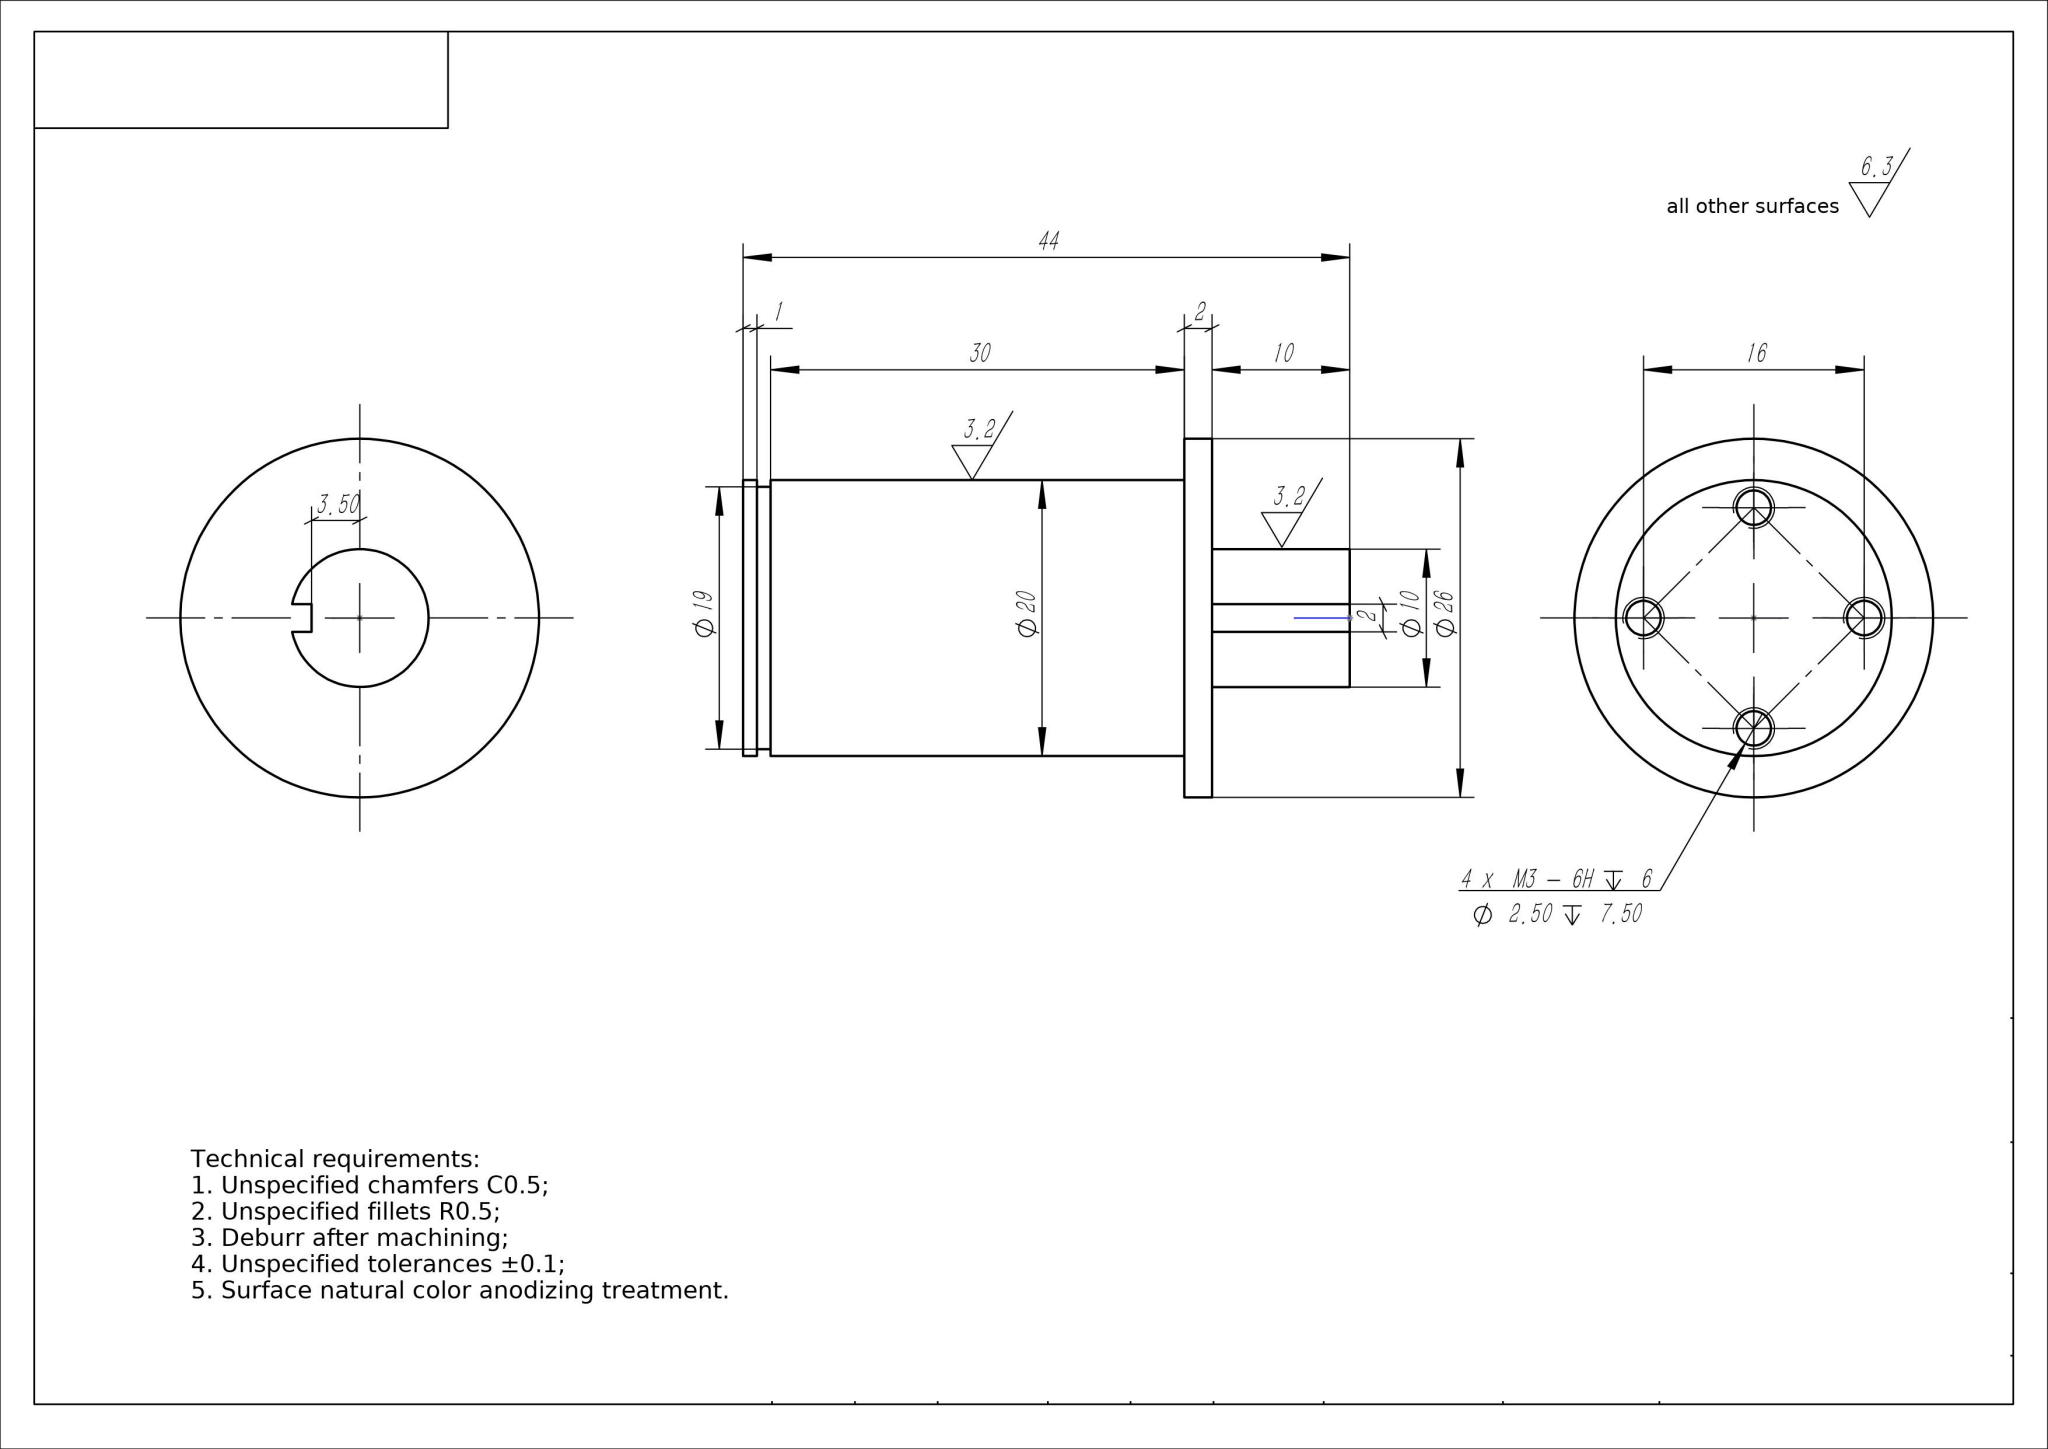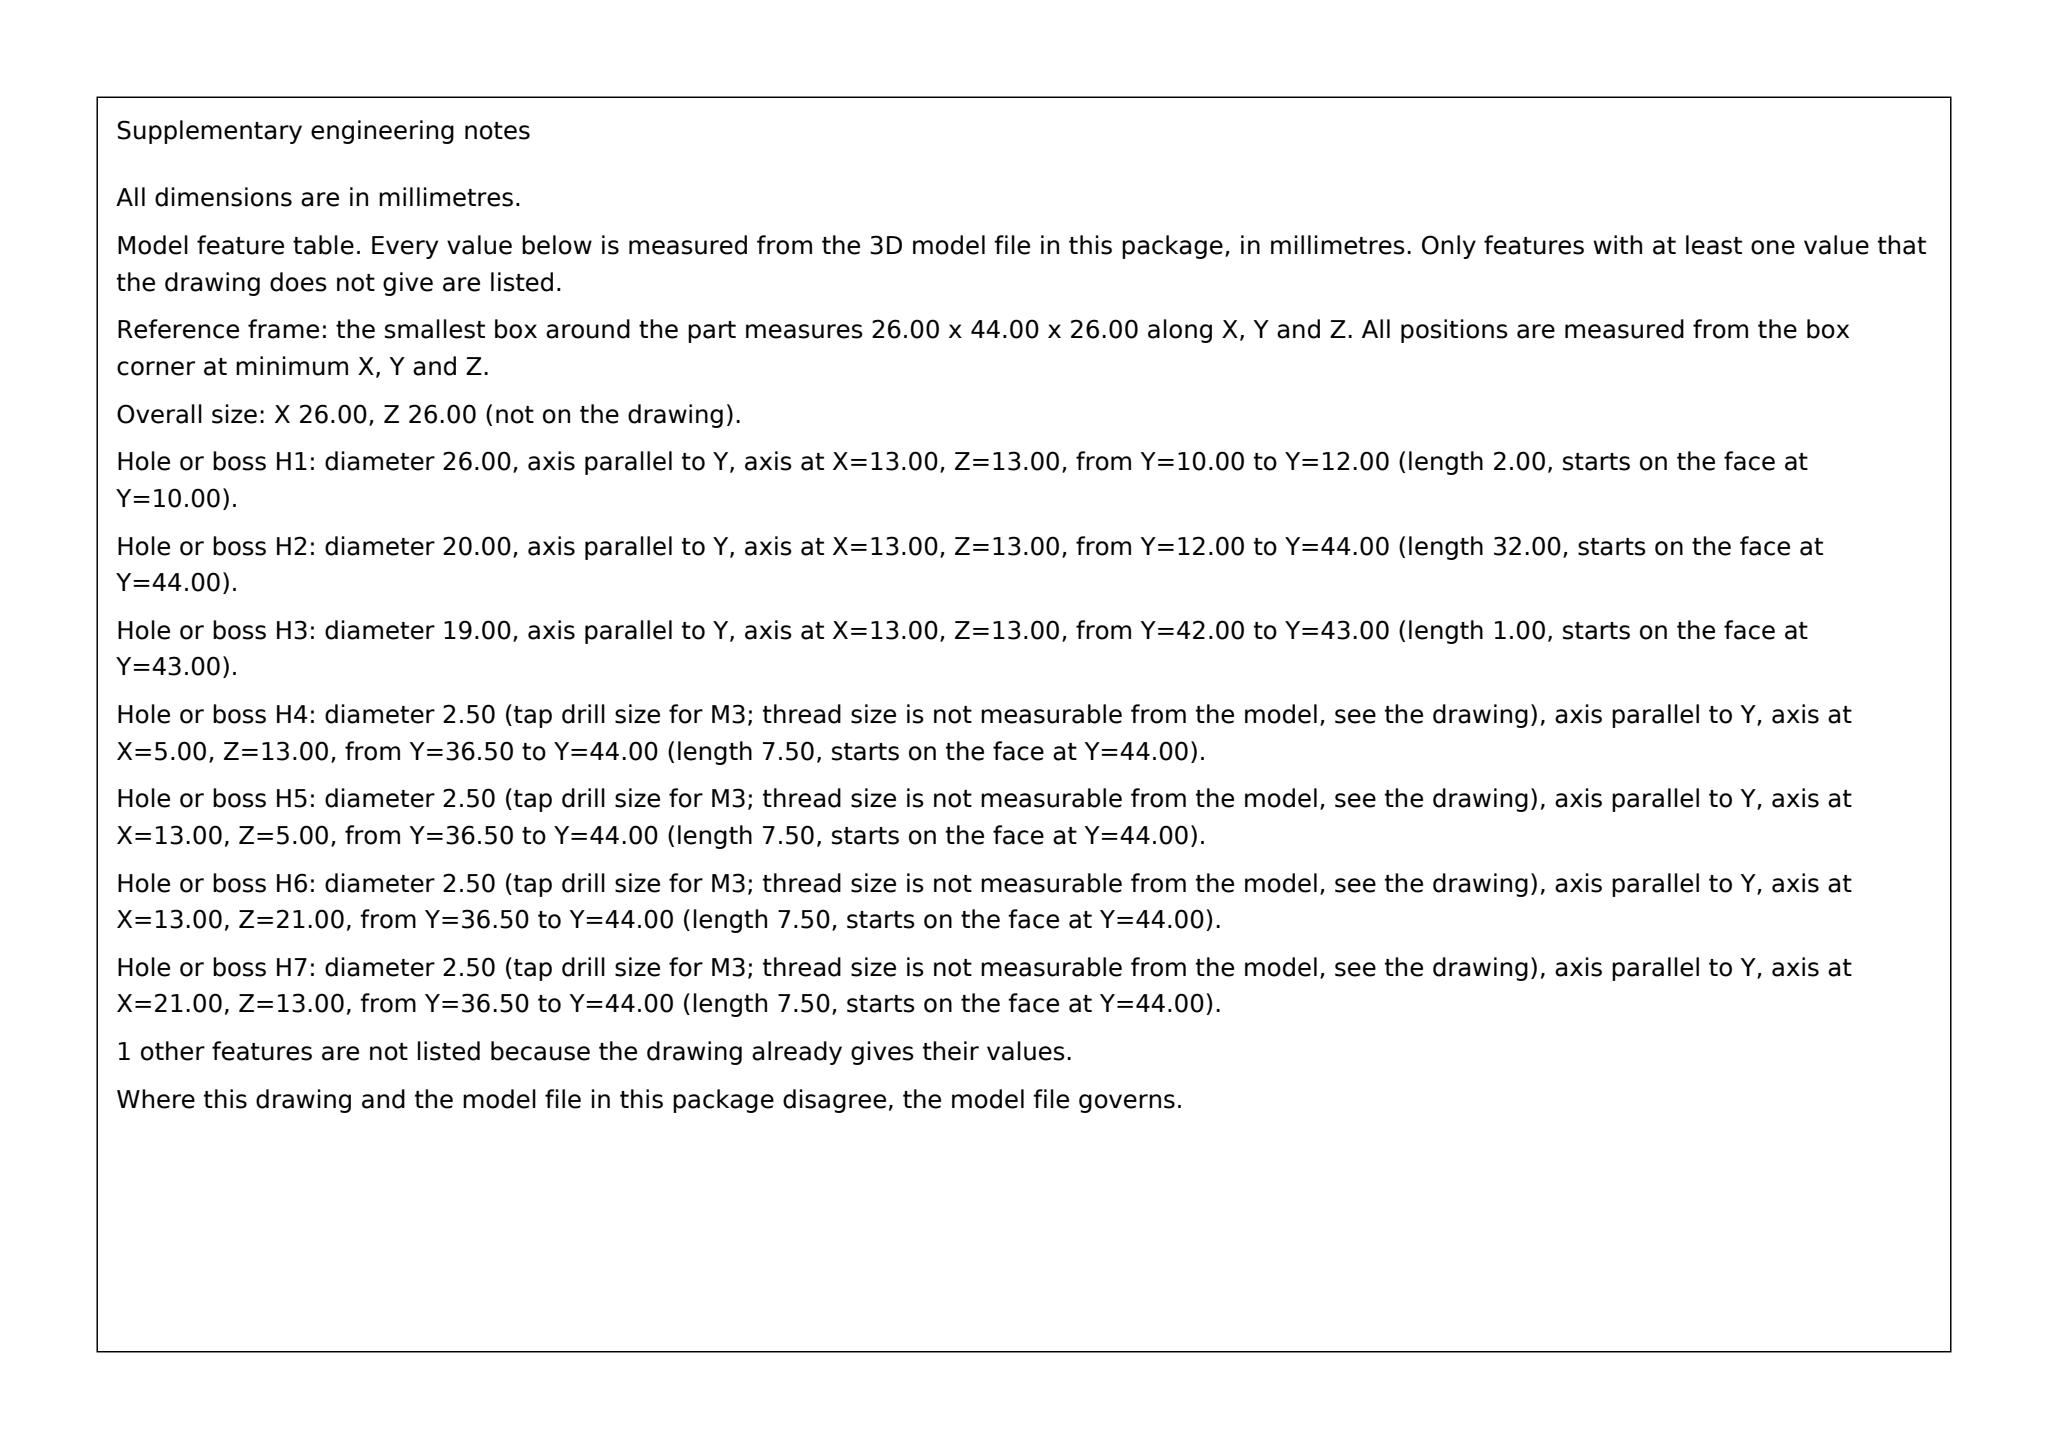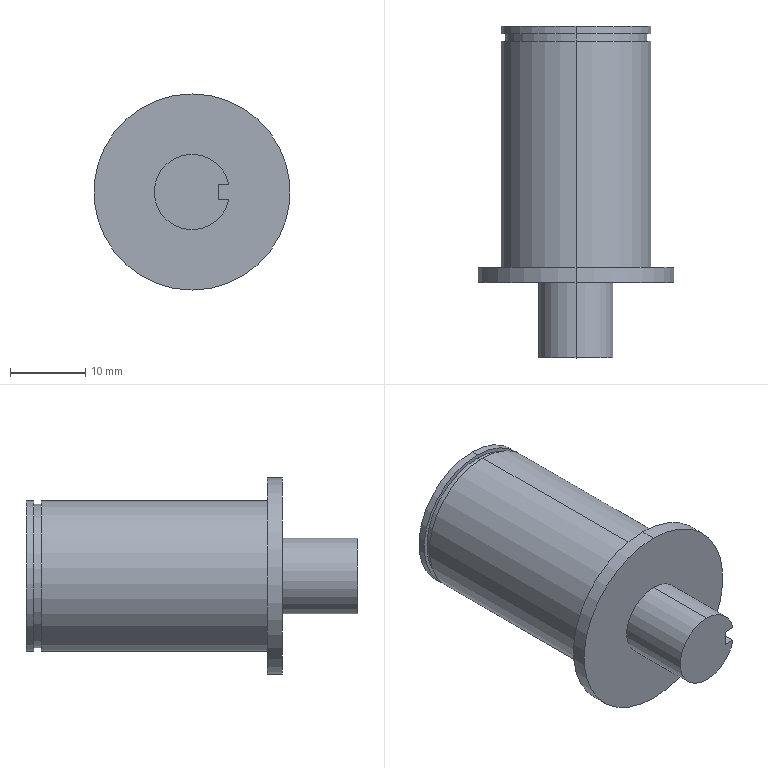Part | SolidWorks | mm | 1 solid | 36 faces | box 26 x 44 x 26 mm | volume 11688 mm3 | cylinder 19 | plane 9 | cone 8 | commonest cylinder face diameters 2.5 x8 20 x4 10 x3 19 x2 26 x2
build123d program:
from build123d import *

# Parameters (mm, degrees)
SKETCH1_R             = 5
BOSS_EXTRUDE1_DEPTH   = 10
SKETCH2_R             = 13
BOSS_EXTRUDE2_DEPTH   = 2
SKETCH4_R             = 10
BOSS_EXTRUDE3_DEPTH   = 32
M3_TAPPED_HOLE1_D     = 2.5
M3_TAPPED_HOLE1_DEPTH = 7.5
M3_TAPPED_HOLE1_TIP   = 0.7511
SKETCH9_W             = 1
SKETCH9_H             = 1
SKETCH10_W            = 3
SKETCH10_H            = 2
CUT_EXTRUDE1_DEPTH    = 10


with BuildPart() as part:
    # Sketch1 → Boss-Extrude1 (new body)
    with BuildSketch(Plane(origin=(0, 0, 0), x_dir=(1, 0, 0), z_dir=(0, 1, 0))):
        with Locations(Location((0, 0, 0), (0, 0, 270))):
            Circle(SKETCH1_R)
    extrude(amount=BOSS_EXTRUDE1_DEPTH)

    # Sketch2 → Boss-Extrude2 (add)
    with BuildSketch(Plane(origin=(0, 10, 0), x_dir=(1, 0, 0), z_dir=(0, 1, 0))):
        with Locations(Location((0, 0, 0), (0, 0, 270))):
            Circle(SKETCH2_R)
    extrude(amount=BOSS_EXTRUDE2_DEPTH)

    # Sketch4 → Boss-Extrude3 (add)
    with BuildSketch(Plane(origin=(0, 12, 0), x_dir=(1, 0, 0), z_dir=(0, 1, 0))):
        with Locations(Location((0, 0, 0), (0, 0, 270))):
            Circle(SKETCH4_R)
    extrude(amount=BOSS_EXTRUDE3_DEPTH)

    # M3 Tapped Hole1
    with Locations(Plane(origin=(0, 44, 0), x_dir=(1, 0, 0), z_dir=(0, 1, 0))):
        with Locations((0, 8), (8, 0), (0, -8), (-8, 0)):
            Hole(M3_TAPPED_HOLE1_D / 2, depth=M3_TAPPED_HOLE1_DEPTH)
            with Locations((0, 0, -(M3_TAPPED_HOLE1_DEPTH + M3_TAPPED_HOLE1_TIP / 2))):  # 118° drill point
                Cone(0, M3_TAPPED_HOLE1_D / 2, M3_TAPPED_HOLE1_TIP, mode=Mode.SUBTRACT)

    # Sketch9 → Cut-Revolve1 (revolve, cut)
    with BuildSketch(Plane.XY, mode=Mode.PRIVATE) as cut_revolve1_sk:
        with Locations((10, 42.5)):
            Rectangle(SKETCH9_W, SKETCH9_H)
    revolve(cut_revolve1_sk.sketch.rotate(Axis((0, 44, 0), (0, -1, 0)), 90), axis=Axis((0, 44, 0), (0, -1, 0)), mode=Mode.SUBTRACT)

    # Sketch10 → Cut-Extrude1 (cut)
    with BuildSketch(Plane.XZ):
        with Locations((5, 0)):
            Rectangle(SKETCH10_W, SKETCH10_H)
    extrude(amount=-CUT_EXTRUDE1_DEPTH, mode=Mode.SUBTRACT)


solid = part.part